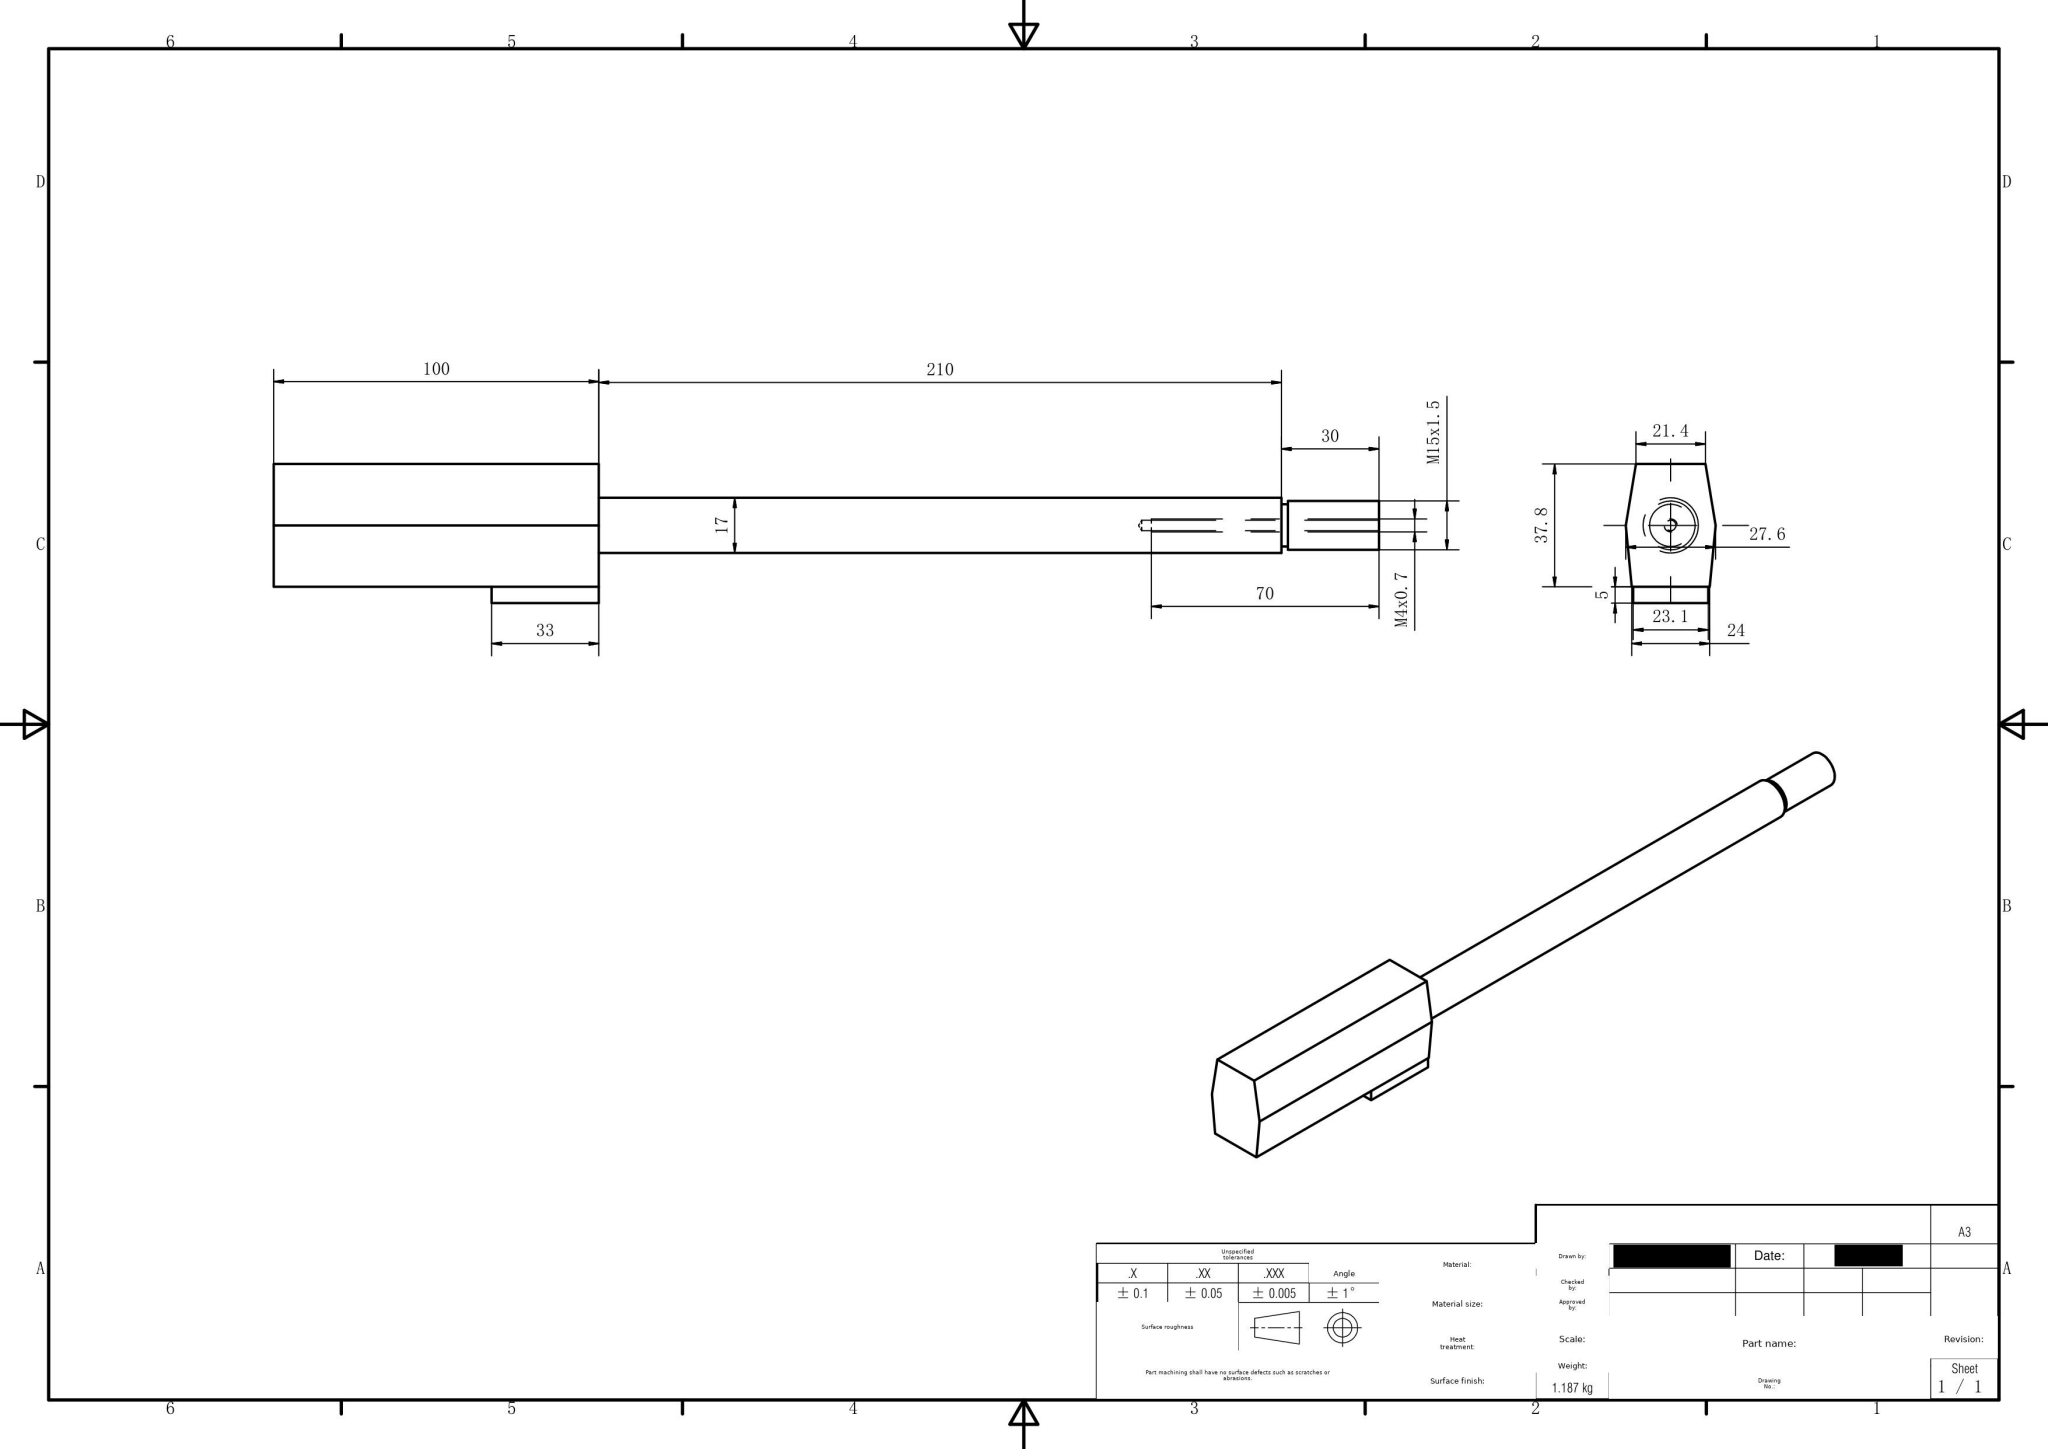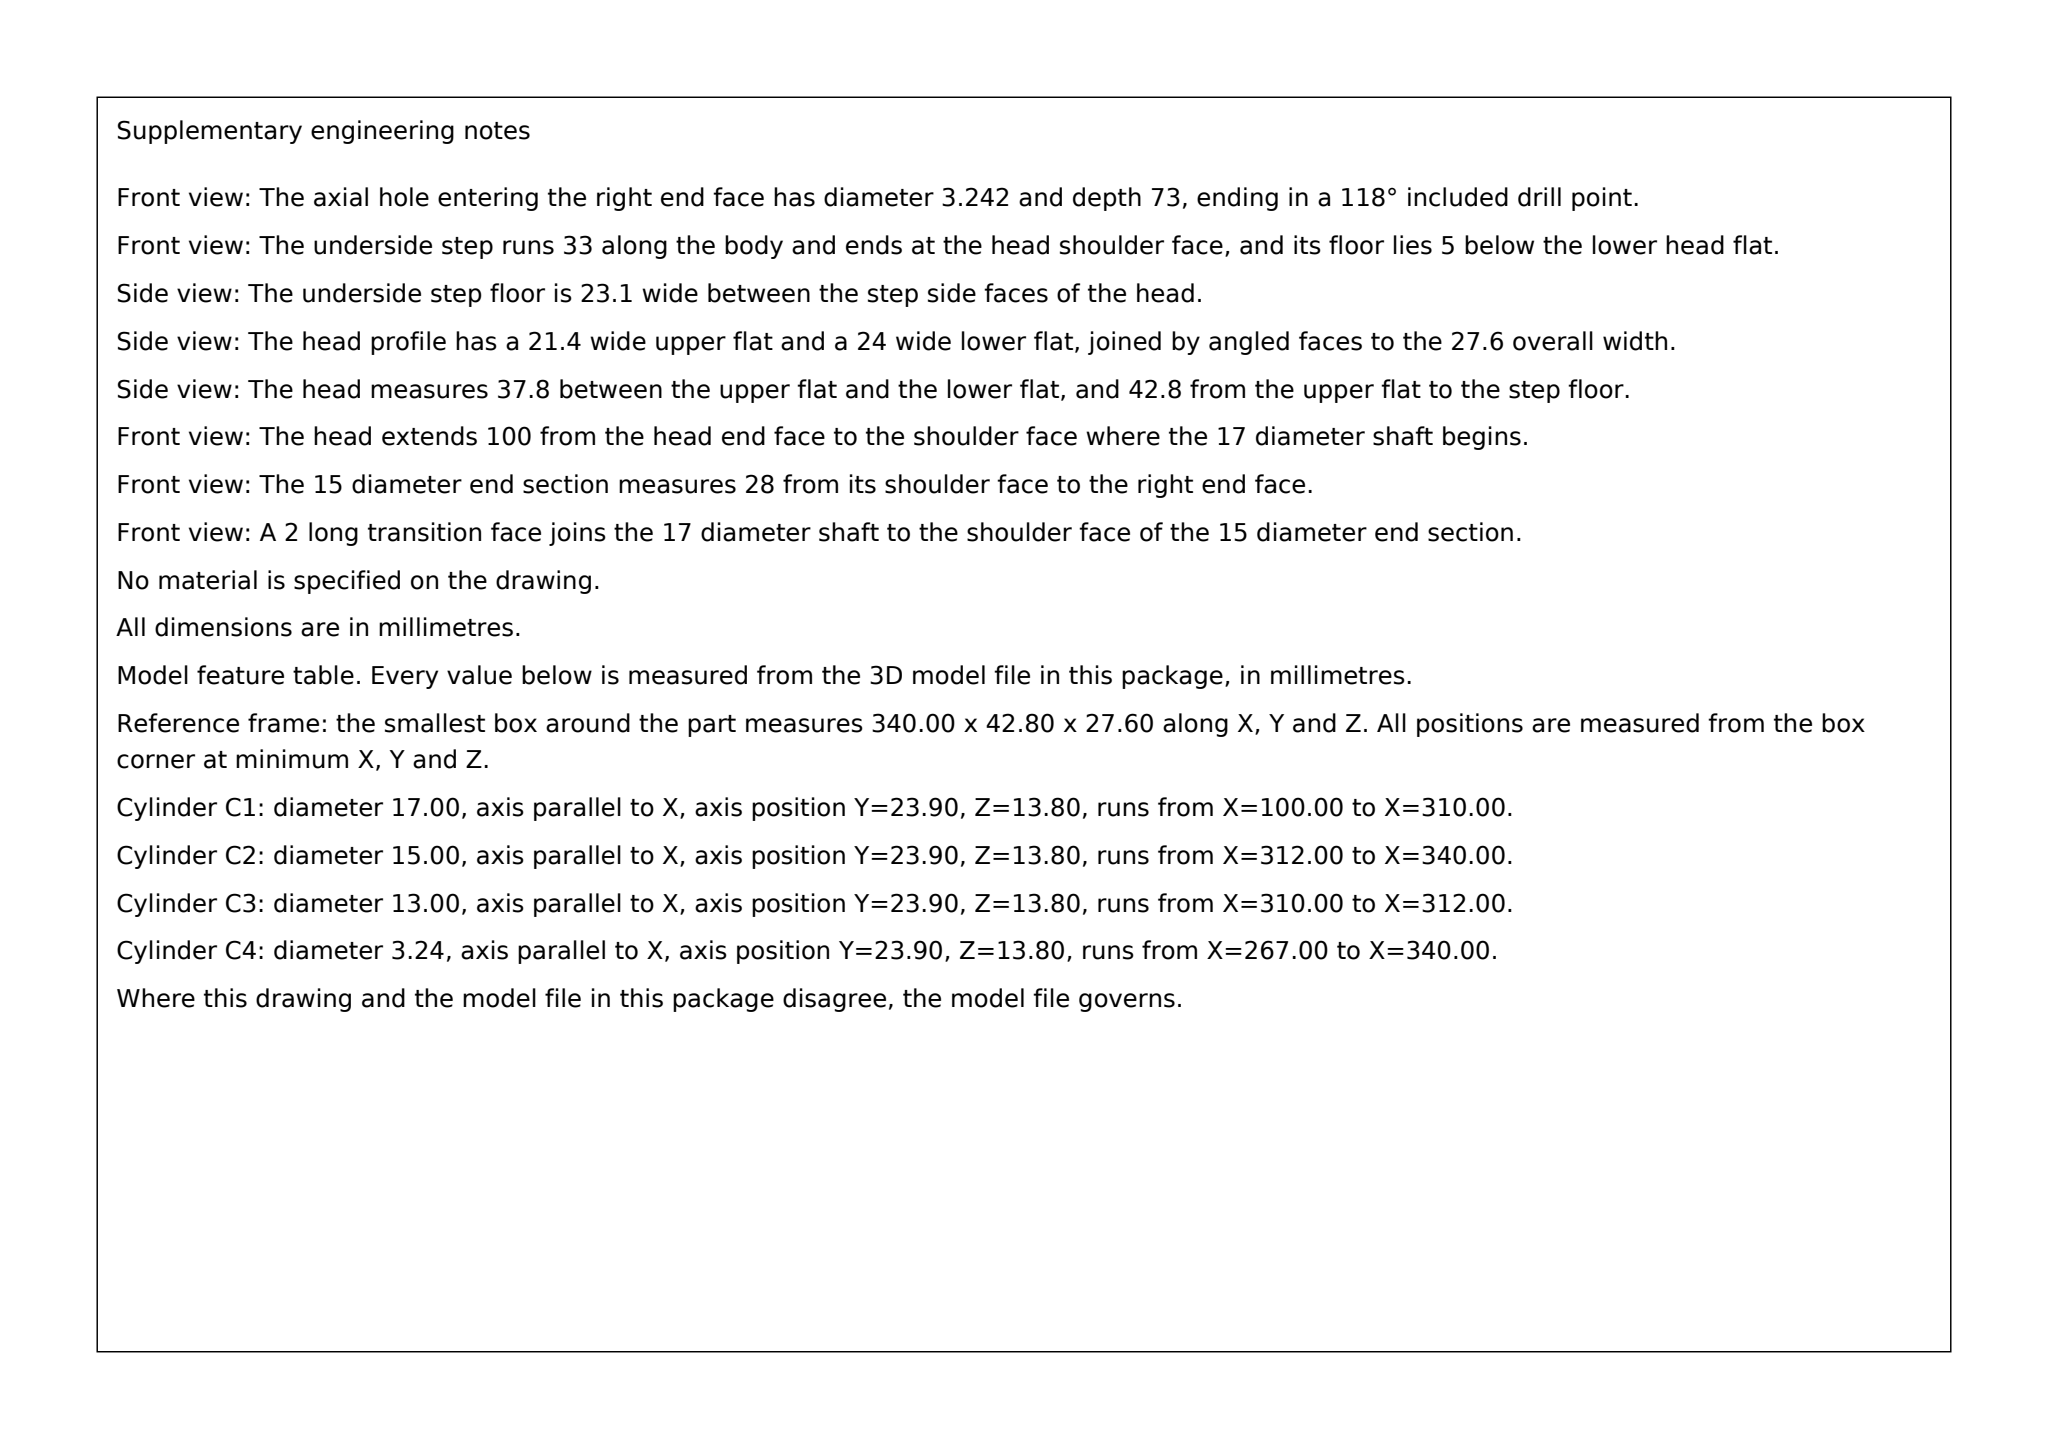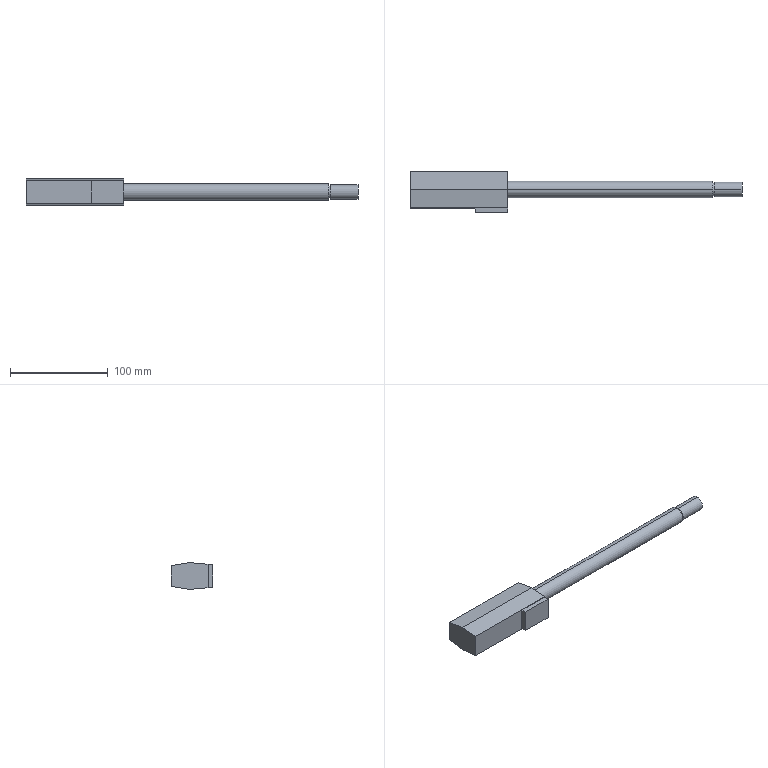Part | SolidWorks | mm | 1 solid | 25 faces | box 340 x 42.8 x 27.6 mm | volume 151152 mm3 | plane 15 | cylinder 8 | cone 2 | commonest cylinder face diameters 3.242 x2 13 x2 15 x2 17 x2
Drawing notes:
Ø13 x 2 WIDE RELIEF, FROM 310 TO 312 FROM HEAD BUTT END FACE (LH) | from the solid: cylinders[13.0,x,len 2.0]; axis_planes x=310.0 and x=312.0
HEAD OVERALL HEIGHT 42.8 FROM BOTTOM FACE (Y=0) TO TOP FACE (Y=42.8); SHAFT AXIS AT Y=23.9, Z=13.8 | from the solid: axis_planes y=0.0 and y=42.8; cylinders dia 17/15/13/3.242 axis x at [y=23.9, z=13.8]
HEAD BOTTOM STEP: 23.1 WIDE (Z=2.3 TO 25.4, SYMM ABOUT SHAFT AXIS Z=13.8) X 5 HIGH (Y=0 TO 5) X 33 LONG (X=67 TO 100 FROM HEAD BUTT END FACE X=0); 24 IS HEAD WIDTH AT Y=5 | from the solid: axis_planes y=0.0 extent x 67-100, z 2.3-25.4; z=2.3 and z=25.4 planes extent x 67-100, y 0-5; axis_plane x=67.0 extent y 0-5, z 2.3-25.4
TAP DRILL Ø3.242 THRU DEPTH 73 FROM THREADED END FACE X=340 (DRILL BOTTOM X=267, 118° POINT TO X=266), ON SHAFT AXIS Y=23.9 Z=13.8 | from the solid: hole/bore dia 3.24 axis x from 267.0 to 340.0 at [null,23.9,13.8]; cones included_angle 118.0 ref_dia 3.24 bbox_from [266.0,...]
M4x0.7 THD DP 70 FULL, TAP DRILL Ø3.24 DP 73 FROM M15x1.5 END | from the solid: hole/bore dia 3.24 along x from 267 to 340 (73 deep from end face x=340, which is the M15x1.5 end); 118° drill point at x=266-267; thread depth per existing 70 dim from same end face
build123d program:
from build123d import *

# Parameters (mm, degrees)
BOSS_EXTRUDE1_DEPTH      = 100
SKETCH2_W                = 33
SKETCH2_H                = 23.1
BOSS_EXTRUDE2_DEPTH      = 5
DRAFT1_ANGLE             = 5.44
M3_CLEARANCE_HOLE1_D     = 3.242
M3_CLEARANCE_HOLE1_DEPTH = 73
M3_CLEARANCE_HOLE1_TIP   = 0.974


with BuildPart() as part:
    # Sketch1 → Boss-Extrude1 (new body)
    with BuildSketch(Plane(origin=(100, 0, 0), x_dir=(0, 0, -1), z_dir=(1, 0, 0))):
        Polygon((-12, 10.974), (-12, -18.9), (12, -18.9), (12, 10.974), (10.7, 18.9), (-10.7, 18.9), align=None)
    extrude(amount=-BOSS_EXTRUDE1_DEPTH)

    # Sketch2 → Boss-Extrude2 (add)
    with BuildSketch(Plane.XZ.offset(18.9)):
        with Locations((83.5, 0)):
            Rectangle(SKETCH2_W, SKETCH2_H)
    extrude(amount=BOSS_EXTRUDE2_DEPTH)

    # Draft1
    draft1_faces = [part.faces().sort_by_distance(p)[0] for p in [
        (50, -3.963, 12),
        (50, -3.963, -12),
    ]]
    draft(draft1_faces, Plane(origin=(0, -18.9, 12), x_dir=(0, 0, -1), z_dir=(0, -1, 0)), DRAFT1_ANGLE)

    # Sketch3 → Revolve1 (revolve)
    with BuildSketch(Plane.XY, mode=Mode.PRIVATE) as revolve1_sk:
        Polygon((100, 8.5), (100, 0), (340, 0), (340, 7.5), (312, 7.5), (312, 6.5), (310, 6.5), (310, 8.5), align=None)
    revolve(revolve1_sk.sketch.rotate(Axis((100, 0, 0), (1, 0, 0)), 270), axis=Axis((100, 0, 0), (1, 0, 0)))

    # M3 Clearance Hole1
    with Locations(Plane(origin=(340, 0, 0), x_dir=(0, 0, -1), z_dir=(1, 0, 0))):
        with Locations((0, 0)):
            Hole(M3_CLEARANCE_HOLE1_D / 2, depth=M3_CLEARANCE_HOLE1_DEPTH)
            with Locations((0, 0, -(M3_CLEARANCE_HOLE1_DEPTH + M3_CLEARANCE_HOLE1_TIP / 2))):  # 118° drill point
                Cone(0, M3_CLEARANCE_HOLE1_D / 2, M3_CLEARANCE_HOLE1_TIP, mode=Mode.SUBTRACT)


solid = part.part
STEP:
#1=CARTESIAN_POINT('',(267.,0.,1.621));
#2=VERTEX_POINT('',#1);
#3=CARTESIAN_POINT('',(267.,0.,-1.621));
#4=VERTEX_POINT('',#3);
#5=CARTESIAN_POINT('',(267.,0.,0.));
#6=DIRECTION('',(1.,0.,0.));
#7=DIRECTION('',(0.,0.,-1.));
#8=AXIS2_PLACEMENT_3D('',#5,#6,#7);
#9=CIRCLE('',#8,1.621);
#10=EDGE_CURVE('',#2,#4,#9,.T.);
#11=ORIENTED_EDGE('',*,*,#10,.F.);
#12=CARTESIAN_POINT('',(340.,0.,1.621));
#13=VERTEX_POINT('',#12);
#14=CARTESIAN_POINT('',(340.,0.,1.621));
#15=DIRECTION('',(1.,0.,0.));
#16=VECTOR('',#15,1000.);
#17=LINE('',#14,#16);
#18=EDGE_CURVE('',#2,#13,#17,.T.);
#19=ORIENTED_EDGE('',*,*,#18,.T.);
#20=CARTESIAN_POINT('',(340.,0.,-1.621));
#21=VERTEX_POINT('',#20);
#22=CARTESIAN_POINT('',(340.,0.,0.));
#23=DIRECTION('',(1.,0.,0.));
#24=DIRECTION('',(0.,0.,-1.));
#25=AXIS2_PLACEMENT_3D('',#22,#23,#24);
#26=CIRCLE('',#25,1.621);
#27=EDGE_CURVE('',#13,#21,#26,.T.);
#28=ORIENTED_EDGE('',*,*,#27,.T.);
#29=CARTESIAN_POINT('',(340.,0.,-1.621));
#30=DIRECTION('',(1.,0.,0.));
#31=VECTOR('',#30,1000.);
#32=LINE('',#29,#31);
#33=EDGE_CURVE('',#4,#21,#32,.T.);
#34=ORIENTED_EDGE('',*,*,#33,.F.);
#35=EDGE_LOOP('',(#11,#19,#28,#34));
#36=FACE_OUTER_BOUND('',#35,.T.);
#37=CARTESIAN_POINT('',(340.,0.,0.));
#38=DIRECTION('',(1.,0.,0.));
#39=DIRECTION('',(0.,0.,-1.));
#40=AXIS2_PLACEMENT_3D('',#37,#38,#39);
#41=CYLINDRICAL_SURFACE('',#40,1.621);
#42=ADVANCED_FACE('',(#36),#41,.F.);
#43=CARTESIAN_POINT('',(266.026,-0.,0.));
#44=VERTEX_POINT('',#43);
#45=CARTESIAN_POINT('',(267.,0.,-1.621));
#46=DIRECTION('',(0.515,0.,-0.8572));
#47=VECTOR('',#46,1000.);
#48=LINE('',#45,#47);
#49=EDGE_CURVE('',#44,#4,#48,.T.);
#50=ORIENTED_EDGE('',*,*,#49,.F.);
#51=CARTESIAN_POINT('',(267.,0.,1.621));
#52=DIRECTION('',(0.515,0.,0.8572));
#53=VECTOR('',#52,1000.);
#54=LINE('',#51,#53);
#55=EDGE_CURVE('',#44,#2,#54,.T.);
#56=ORIENTED_EDGE('',*,*,#55,.T.);
#57=ORIENTED_EDGE('',*,*,#10,.T.);
#58=EDGE_LOOP('',(#50,#56,#57));
#59=FACE_OUTER_BOUND('',#58,.T.);
#60=CARTESIAN_POINT('',(267.,0.,0.));
#61=DIRECTION('',(1.,0.,0.));
#62=DIRECTION('',(0.,0.,-1.));
#63=AXIS2_PLACEMENT_3D('',#60,#61,#62);
#64=CONICAL_SURFACE('',#63,1.621,1.03);
#65=ADVANCED_FACE('',(#59),#64,.F.);
#66=CARTESIAN_POINT('',(310.,0.,-6.5));
#67=VERTEX_POINT('',#66);
#68=CARTESIAN_POINT('',(310.,0.,6.5));
#69=VERTEX_POINT('',#68);
#70=CARTESIAN_POINT('',(310.,0.,0.));
#71=DIRECTION('',(1.,0.,0.));
#72=DIRECTION('',(0.,0.,-1.));
#73=AXIS2_PLACEMENT_3D('',#70,#71,#72);
#74=CIRCLE('',#73,6.5);
#75=EDGE_CURVE('',#67,#69,#74,.T.);
#76=ORIENTED_EDGE('',*,*,#75,.T.);
#77=CARTESIAN_POINT('',(312.,0.,6.5));
#78=VERTEX_POINT('',#77);
#79=CARTESIAN_POINT('',(100.,0.,6.5));
#80=DIRECTION('',(1.,0.,0.));
#81=VECTOR('',#80,1000.);
#82=LINE('',#79,#81);
#83=EDGE_CURVE('',#69,#78,#82,.T.);
#84=ORIENTED_EDGE('',*,*,#83,.T.);
#85=CARTESIAN_POINT('',(312.,0.,-6.5));
#86=VERTEX_POINT('',#85);
#87=CARTESIAN_POINT('',(312.,0.,0.));
#88=DIRECTION('',(1.,0.,0.));
#89=DIRECTION('',(0.,0.,-1.));
#90=AXIS2_PLACEMENT_3D('',#87,#88,#89);
#91=CIRCLE('',#90,6.5);
#92=EDGE_CURVE('',#86,#78,#91,.T.);
#93=ORIENTED_EDGE('',*,*,#92,.F.);
#94=CARTESIAN_POINT('',(100.,0.,-6.5));
#95=DIRECTION('',(1.,0.,0.));
#96=VECTOR('',#95,1000.);
#97=LINE('',#94,#96);
#98=EDGE_CURVE('',#67,#86,#97,.T.);
#99=ORIENTED_EDGE('',*,*,#98,.F.);
#100=EDGE_LOOP('',(#76,#84,#93,#99));
#101=FACE_OUTER_BOUND('',#100,.T.);
#102=CARTESIAN_POINT('',(100.,0.,0.));
#103=DIRECTION('',(1.,0.,0.));
#104=DIRECTION('',(0.,0.,-1.));
#105=AXIS2_PLACEMENT_3D('',#102,#103,#104);
#106=CYLINDRICAL_SURFACE('',#105,6.5);
#107=ADVANCED_FACE('',(#101),#106,.T.);
#108=CARTESIAN_POINT('',(312.,0.,-7.5));
#109=VERTEX_POINT('',#108);
#110=CARTESIAN_POINT('',(312.,0.,7.5));
#111=VERTEX_POINT('',#110);
#112=CARTESIAN_POINT('',(312.,0.,0.));
#113=DIRECTION('',(1.,0.,0.));
#114=DIRECTION('',(0.,0.,-1.));
#115=AXIS2_PLACEMENT_3D('',#112,#113,#114);
#116=CIRCLE('',#115,7.5);
#117=EDGE_CURVE('',#109,#111,#116,.T.);
#118=ORIENTED_EDGE('',*,*,#117,.T.);
#119=CARTESIAN_POINT('',(340.,0.,7.5));
#120=VERTEX_POINT('',#119);
#121=CARTESIAN_POINT('',(100.,0.,7.5));
#122=DIRECTION('',(1.,0.,0.));
#123=VECTOR('',#122,1000.);
#124=LINE('',#121,#123);
#125=EDGE_CURVE('',#111,#120,#124,.T.);
#126=ORIENTED_EDGE('',*,*,#125,.T.);
#127=CARTESIAN_POINT('',(340.,0.,-7.5));
#128=VERTEX_POINT('',#127);
#129=CARTESIAN_POINT('',(340.,0.,0.));
#130=DIRECTION('',(1.,0.,0.));
#131=DIRECTION('',(0.,0.,-1.));
#132=AXIS2_PLACEMENT_3D('',#129,#130,#131);
#133=CIRCLE('',#132,7.5);
#134=EDGE_CURVE('',#128,#120,#133,.T.);
#135=ORIENTED_EDGE('',*,*,#134,.F.);
#136=CARTESIAN_POINT('',(100.,0.,-7.5));
#137=DIRECTION('',(1.,0.,0.));
#138=VECTOR('',#137,1000.);
#139=LINE('',#136,#138);
#140=EDGE_CURVE('',#109,#128,#139,.T.);
#141=ORIENTED_EDGE('',*,*,#140,.F.);
#142=EDGE_LOOP('',(#118,#126,#135,#141));
#143=FACE_OUTER_BOUND('',#142,.T.);
#144=CARTESIAN_POINT('',(100.,0.,0.));
#145=DIRECTION('',(1.,0.,0.));
#146=DIRECTION('',(0.,0.,-1.));
#147=AXIS2_PLACEMENT_3D('',#144,#145,#146);
#148=CYLINDRICAL_SURFACE('',#147,7.5);
#149=ADVANCED_FACE('',(#143),#148,.T.);
#150=CARTESIAN_POINT('',(100.,0.,-8.5));
#151=VERTEX_POINT('',#150);
#152=CARTESIAN_POINT('',(100.,0.,8.5));
#153=VERTEX_POINT('',#152);
#154=CARTESIAN_POINT('',(100.,0.,0.));
#155=DIRECTION('',(1.,0.,0.));
#156=DIRECTION('',(0.,0.,-1.));
#157=AXIS2_PLACEMENT_3D('',#154,#155,#156);
#158=CIRCLE('',#157,8.5);
#159=EDGE_CURVE('',#151,#153,#158,.T.);
#160=ORIENTED_EDGE('',*,*,#159,.T.);
#161=CARTESIAN_POINT('',(310.,0.,8.5));
#162=VERTEX_POINT('',#161);
#163=CARTESIAN_POINT('',(100.,0.,8.5));
#164=DIRECTION('',(1.,0.,0.));
#165=VECTOR('',#164,1000.);
#166=LINE('',#163,#165);
#167=EDGE_CURVE('',#153,#162,#166,.T.);
#168=ORIENTED_EDGE('',*,*,#167,.T.);
#169=CARTESIAN_POINT('',(310.,0.,-8.5));
#170=VERTEX_POINT('',#169);
#171=CARTESIAN_POINT('',(310.,0.,0.));
#172=DIRECTION('',(1.,0.,0.));
#173=DIRECTION('',(0.,0.,-1.));
#174=AXIS2_PLACEMENT_3D('',#171,#172,#173);
#175=CIRCLE('',#174,8.5);
#176=EDGE_CURVE('',#170,#162,#175,.T.);
#177=ORIENTED_EDGE('',*,*,#176,.F.);
#178=CARTESIAN_POINT('',(100.,0.,-8.5));
#179=DIRECTION('',(1.,0.,0.));
#180=VECTOR('',#179,1000.);
#181=LINE('',#178,#180);
#182=EDGE_CURVE('',#151,#170,#181,.T.);
#183=ORIENTED_EDGE('',*,*,#182,.F.);
#184=EDGE_LOOP('',(#160,#168,#177,#183));
#185=FACE_OUTER_BOUND('',#184,.T.);
#186=CARTESIAN_POINT('',(100.,0.,0.));
#187=DIRECTION('',(1.,0.,0.));
#188=DIRECTION('',(0.,0.,-1.));
#189=AXIS2_PLACEMENT_3D('',#186,#187,#188);
#190=CYLINDRICAL_SURFACE('',#189,8.5);
#191=ADVANCED_FACE('',(#185),#190,.T.);
#192=CARTESIAN_POINT('',(100.,18.9,10.7));
#193=VERTEX_POINT('',#192);
#194=CARTESIAN_POINT('',(100.,-0.,13.8));
#195=VERTEX_POINT('',#194);
#196=CARTESIAN_POINT('',(100.,18.9,10.7));
#197=DIRECTION('',(0.,-0.9868,0.1619));
#198=VECTOR('',#197,1000.);
#199=LINE('',#196,#198);
#200=EDGE_CURVE('',#193,#195,#199,.T.);
#201=ORIENTED_EDGE('',*,*,#200,.F.);
#202=CARTESIAN_POINT('',(0.,18.9,10.7));
#203=VERTEX_POINT('',#202);
#204=CARTESIAN_POINT('',(0.,18.9,10.7));
#205=DIRECTION('',(1.,0.,0.));
#206=VECTOR('',#205,1000.);
#207=LINE('',#204,#206);
#208=EDGE_CURVE('',#203,#193,#207,.T.);
#209=ORIENTED_EDGE('',*,*,#208,.F.);
#210=CARTESIAN_POINT('',(0.,-0.,13.8));
#211=VERTEX_POINT('',#210);
#212=CARTESIAN_POINT('',(0.,18.9,10.7));
#213=DIRECTION('',(0.,-0.9868,0.1619));
#214=VECTOR('',#213,1000.);
#215=LINE('',#212,#214);
#216=EDGE_CURVE('',#203,#211,#215,.T.);
#217=ORIENTED_EDGE('',*,*,#216,.T.);
#218=CARTESIAN_POINT('',(0.,-0.,13.8));
#219=DIRECTION('',(1.,0.,0.));
#220=VECTOR('',#219,1000.);
#221=LINE('',#218,#220);
#222=EDGE_CURVE('',#211,#195,#221,.T.);
#223=ORIENTED_EDGE('',*,*,#222,.T.);
#224=EDGE_LOOP('',(#201,#209,#217,#223));
#225=FACE_OUTER_BOUND('',#224,.T.);
#226=CARTESIAN_POINT('',(0.,18.9,10.7));
#227=DIRECTION('',(0.,0.1619,0.9868));
#228=DIRECTION('',(0.,-0.9868,0.1619));
#229=AXIS2_PLACEMENT_3D('',#226,#227,#228);
#230=PLANE('',#229);
#231=ADVANCED_FACE('',(#225),#230,.T.);
#232=CARTESIAN_POINT('',(100.,18.9,-10.7));
#233=VERTEX_POINT('',#232);
#234=CARTESIAN_POINT('',(100.,18.9,-10.7));
#235=DIRECTION('',(0.,-0.,1.));
#236=VECTOR('',#235,1000.);
#237=LINE('',#234,#236);
#238=EDGE_CURVE('',#233,#193,#237,.T.);
#239=ORIENTED_EDGE('',*,*,#238,.F.);
#240=CARTESIAN_POINT('',(0.,18.9,-10.7));
#241=VERTEX_POINT('',#240);
#242=CARTESIAN_POINT('',(0.,18.9,-10.7));
#243=DIRECTION('',(1.,0.,0.));
#244=VECTOR('',#243,1000.);
#245=LINE('',#242,#244);
#246=EDGE_CURVE('',#241,#233,#245,.T.);
#247=ORIENTED_EDGE('',*,*,#246,.F.);
#248=CARTESIAN_POINT('',(0.,18.9,-10.7));
#249=DIRECTION('',(0.,-0.,1.));
#250=VECTOR('',#249,1000.);
#251=LINE('',#248,#250);
#252=EDGE_CURVE('',#241,#203,#251,.T.);
#253=ORIENTED_EDGE('',*,*,#252,.T.);
#254=ORIENTED_EDGE('',*,*,#208,.T.);
#255=EDGE_LOOP('',(#239,#247,#253,#254));
#256=FACE_OUTER_BOUND('',#255,.T.);
#257=CARTESIAN_POINT('',(0.,18.9,-10.7));
#258=DIRECTION('',(0.,1.,0.));
#259=DIRECTION('',(0.,-0.,1.));
#260=AXIS2_PLACEMENT_3D('',#257,#258,#259);
#261=PLANE('',#260);
#262=ADVANCED_FACE('',(#256),#261,.T.);
#263=CARTESIAN_POINT('',(100.,-0.,-13.8));
#264=VERTEX_POINT('',#263);
#265=CARTESIAN_POINT('',(100.,10.974,-12.));
#266=DIRECTION('',(0.,0.9868,0.1619));
#267=VECTOR('',#266,1000.);
#268=LINE('',#265,#267);
#269=EDGE_CURVE('',#264,#233,#268,.T.);
#270=ORIENTED_EDGE('',*,*,#269,.F.);
#271=CARTESIAN_POINT('',(0.,-0.,-13.8));
#272=VERTEX_POINT('',#271);
#273=CARTESIAN_POINT('',(0.,-0.,-13.8));
#274=DIRECTION('',(1.,0.,0.));
#275=VECTOR('',#274,1000.);
#276=LINE('',#273,#275);
#277=EDGE_CURVE('',#272,#264,#276,.T.);
#278=ORIENTED_EDGE('',*,*,#277,.F.);
#279=CARTESIAN_POINT('',(0.,10.974,-12.));
#280=DIRECTION('',(0.,0.9868,0.1619));
#281=VECTOR('',#280,1000.);
#282=LINE('',#279,#281);
#283=EDGE_CURVE('',#272,#241,#282,.T.);
#284=ORIENTED_EDGE('',*,*,#283,.T.);
#285=ORIENTED_EDGE('',*,*,#246,.T.);
#286=EDGE_LOOP('',(#270,#278,#284,#285));
#287=FACE_OUTER_BOUND('',#286,.T.);
#288=CARTESIAN_POINT('',(0.,10.974,-12.));
#289=DIRECTION('',(0.,0.1619,-0.9868));
#290=DIRECTION('',(0.,0.9868,0.1619));
#291=AXIS2_PLACEMENT_3D('',#288,#289,#290);
#292=PLANE('',#291);
#293=ADVANCED_FACE('',(#287),#292,.T.);
#294=CARTESIAN_POINT('',(100.,-18.9,-12.));
#295=VERTEX_POINT('',#294);
#296=CARTESIAN_POINT('',(100.,-1.302,-13.676));
#297=DIRECTION('',(0.,0.9955,-0.09481));
#298=VECTOR('',#297,1000.);
#299=LINE('',#296,#298);
#300=EDGE_CURVE('',#295,#264,#299,.T.);
#301=ORIENTED_EDGE('',*,*,#300,.F.);
#302=CARTESIAN_POINT('',(0.,-18.9,-12.));
#303=VERTEX_POINT('',#302);
#304=CARTESIAN_POINT('',(0.,-18.9,-12.));
#305=DIRECTION('',(1.,0.,0.));
#306=VECTOR('',#305,1000.);
#307=LINE('',#304,#306);
#308=EDGE_CURVE('',#303,#295,#307,.T.);
#309=ORIENTED_EDGE('',*,*,#308,.F.);
#310=CARTESIAN_POINT('',(0.,-1.302,-13.676));
#311=DIRECTION('',(0.,0.9955,-0.09481));
#312=VECTOR('',#311,1000.);
#313=LINE('',#310,#312);
#314=EDGE_CURVE('',#303,#272,#313,.T.);
#315=ORIENTED_EDGE('',*,*,#314,.T.);
#316=ORIENTED_EDGE('',*,*,#277,.T.);
#317=EDGE_LOOP('',(#301,#309,#315,#316));
#318=FACE_OUTER_BOUND('',#317,.T.);
#319=CARTESIAN_POINT('',(0.,-18.9,-12.));
#320=DIRECTION('',(0.,-0.09481,-0.9955));
#321=DIRECTION('',(0.,0.9955,-0.09481));
#322=AXIS2_PLACEMENT_3D('',#319,#320,#321);
#323=PLANE('',#322);
#324=ADVANCED_FACE('',(#318),#323,.T.);
#325=CARTESIAN_POINT('',(67.,-18.9,-11.55));
#326=VERTEX_POINT('',#325);
#327=CARTESIAN_POINT('',(100.,-18.9,-11.55));
#328=VERTEX_POINT('',#327);
#329=CARTESIAN_POINT('',(100.,-18.9,-11.55));
#330=DIRECTION('',(1.,0.,0.));
#331=VECTOR('',#330,1000.);
#332=LINE('',#329,#331);
#333=EDGE_CURVE('',#326,#328,#332,.T.);
#334=ORIENTED_EDGE('',*,*,#333,.F.);
#335=CARTESIAN_POINT('',(67.,-18.9,11.55));
#336=VERTEX_POINT('',#335);
#337=CARTESIAN_POINT('',(67.,-18.9,-11.55));
#338=DIRECTION('',(0.,0.,-1.));
#339=VECTOR('',#338,1000.);
#340=LINE('',#337,#339);
#341=EDGE_CURVE('',#336,#326,#340,.T.);
#342=ORIENTED_EDGE('',*,*,#341,.F.);
#343=CARTESIAN_POINT('',(100.,-18.9,11.55));
#344=VERTEX_POINT('',#343);
#345=CARTESIAN_POINT('',(67.,-18.9,11.55));
#346=DIRECTION('',(-1.,0.,0.));
#347=VECTOR('',#346,1000.);
#348=LINE('',#345,#347);
#349=EDGE_CURVE('',#344,#336,#348,.T.);
#350=ORIENTED_EDGE('',*,*,#349,.F.);
#351=CARTESIAN_POINT('',(100.,-18.9,12.));
#352=VERTEX_POINT('',#351);
#353=CARTESIAN_POINT('',(100.,-18.9,12.));
#354=DIRECTION('',(0.,0.,-1.));
#355=VECTOR('',#354,1000.);
#356=LINE('',#353,#355);
#357=EDGE_CURVE('',#352,#344,#356,.T.);
#358=ORIENTED_EDGE('',*,*,#357,.F.);
#359=CARTESIAN_POINT('',(0.,-18.9,12.));
#360=VERTEX_POINT('',#359);
#361=CARTESIAN_POINT('',(0.,-18.9,12.));
#362=DIRECTION('',(1.,0.,0.));
#363=VECTOR('',#362,1000.);
#364=LINE('',#361,#363);
#365=EDGE_CURVE('',#360,#352,#364,.T.);
#366=ORIENTED_EDGE('',*,*,#365,.F.);
#367=CARTESIAN_POINT('',(0.,-18.9,12.));
#368=DIRECTION('',(0.,0.,-1.));
#369=VECTOR('',#368,1000.);
#370=LINE('',#367,#369);
#371=EDGE_CURVE('',#360,#303,#370,.T.);
#372=ORIENTED_EDGE('',*,*,#371,.T.);
#373=ORIENTED_EDGE('',*,*,#308,.T.);
#374=CARTESIAN_POINT('',(100.,-18.9,12.));
#375=DIRECTION('',(0.,0.,-1.));
#376=VECTOR('',#375,1000.);
#377=LINE('',#374,#376);
#378=EDGE_CURVE('',#328,#295,#377,.T.);
#379=ORIENTED_EDGE('',*,*,#378,.F.);
#380=EDGE_LOOP('',(#334,#342,#350,#358,#366,#372,#373,#379));
#381=FACE_OUTER_BOUND('',#380,.T.);
#382=CARTESIAN_POINT('',(0.,-18.9,12.));
#383=DIRECTION('',(0.,-1.,-0.));
#384=DIRECTION('',(0.,0.,-1.));
#385=AXIS2_PLACEMENT_3D('',#382,#383,#384);
#386=PLANE('',#385);
#387=ADVANCED_FACE('',(#381),#386,.T.);
#388=CARTESIAN_POINT('',(100.,-1.302,13.676));
#389=DIRECTION('',(0.,-0.9955,-0.09481));
#390=VECTOR('',#389,1000.);
#391=LINE('',#388,#390);
#392=EDGE_CURVE('',#195,#352,#391,.T.);
#393=ORIENTED_EDGE('',*,*,#392,.F.);
#394=ORIENTED_EDGE('',*,*,#222,.F.);
#395=CARTESIAN_POINT('',(0.,-1.302,13.676));
#396=DIRECTION('',(0.,-0.9955,-0.09481));
#397=VECTOR('',#396,1000.);
#398=LINE('',#395,#397);
#399=EDGE_CURVE('',#211,#360,#398,.T.);
#400=ORIENTED_EDGE('',*,*,#399,.T.);
#401=ORIENTED_EDGE('',*,*,#365,.T.);
#402=EDGE_LOOP('',(#393,#394,#400,#401));
#403=FACE_OUTER_BOUND('',#402,.T.);
#404=CARTESIAN_POINT('',(0.,-18.9,12.));
#405=DIRECTION('',(0.,-0.09481,0.9955));
#406=DIRECTION('',(0.,-0.9955,-0.09481));
#407=AXIS2_PLACEMENT_3D('',#404,#405,#406);
#408=PLANE('',#407);
#409=ADVANCED_FACE('',(#403),#408,.T.);
#410=ORIENTED_EDGE('',*,*,#216,.F.);
#411=ORIENTED_EDGE('',*,*,#252,.F.);
#412=ORIENTED_EDGE('',*,*,#283,.F.);
#413=ORIENTED_EDGE('',*,*,#314,.F.);
#414=ORIENTED_EDGE('',*,*,#371,.F.);
#415=ORIENTED_EDGE('',*,*,#399,.F.);
#416=EDGE_LOOP('',(#410,#411,#412,#413,#414,#415));
#417=FACE_OUTER_BOUND('',#416,.T.);
#418=CARTESIAN_POINT('',(0.,0.,0.));
#419=DIRECTION('',(1.,0.,0.));
#420=DIRECTION('',(0.,0.,-1.));
#421=AXIS2_PLACEMENT_3D('',#418,#419,#420);
#422=PLANE('',#421);
#423=ADVANCED_FACE('',(#417),#422,.F.);
#424=ORIENTED_EDGE('',*,*,#159,.F.);
#425=CARTESIAN_POINT('',(100.,0.,0.));
#426=DIRECTION('',(1.,0.,0.));
#427=DIRECTION('',(0.,0.,-1.));
#428=AXIS2_PLACEMENT_3D('',#425,#426,#427);
#429=CIRCLE('',#428,8.5);
#430=EDGE_CURVE('',#153,#151,#429,.T.);
#431=ORIENTED_EDGE('',*,*,#430,.F.);
#432=EDGE_LOOP('',(#424,#431));
#433=FACE_BOUND('',#432,.T.);
#434=ORIENTED_EDGE('',*,*,#200,.T.);
#435=ORIENTED_EDGE('',*,*,#392,.T.);
#436=ORIENTED_EDGE('',*,*,#357,.T.);
#437=CARTESIAN_POINT('',(100.,-23.9,11.55));
#438=VERTEX_POINT('',#437);
#439=CARTESIAN_POINT('',(100.,-23.9,11.55));
#440=DIRECTION('',(0.,1.,0.));
#441=VECTOR('',#440,1000.);
#442=LINE('',#439,#441);
#443=EDGE_CURVE('',#438,#344,#442,.T.);
#444=ORIENTED_EDGE('',*,*,#443,.F.);
#445=CARTESIAN_POINT('',(100.,-23.9,-11.55));
#446=VERTEX_POINT('',#445);
#447=CARTESIAN_POINT('',(100.,-23.9,11.55));
#448=DIRECTION('',(0.,0.,1.));
#449=VECTOR('',#448,1000.);
#450=LINE('',#447,#449);
#451=EDGE_CURVE('',#446,#438,#450,.T.);
#452=ORIENTED_EDGE('',*,*,#451,.F.);
#453=CARTESIAN_POINT('',(100.,-23.9,-11.55));
#454=DIRECTION('',(0.,1.,0.));
#455=VECTOR('',#454,1000.);
#456=LINE('',#453,#455);
#457=EDGE_CURVE('',#446,#328,#456,.T.);
#458=ORIENTED_EDGE('',*,*,#457,.T.);
#459=ORIENTED_EDGE('',*,*,#378,.T.);
#460=ORIENTED_EDGE('',*,*,#300,.T.);
#461=ORIENTED_EDGE('',*,*,#269,.T.);
#462=ORIENTED_EDGE('',*,*,#238,.T.);
#463=EDGE_LOOP('',(#434,#435,#436,#444,#452,#458,#459,#460,#461,#462));
#464=FACE_OUTER_BOUND('',#463,.T.);
#465=CARTESIAN_POINT('',(100.,0.,0.));
#466=DIRECTION('',(1.,0.,0.));
#467=DIRECTION('',(0.,0.,-1.));
#468=AXIS2_PLACEMENT_3D('',#465,#466,#467);
#469=PLANE('',#468);
#470=ADVANCED_FACE('',(#433,#464),#469,.T.);
#471=ORIENTED_EDGE('',*,*,#333,.T.);
#472=ORIENTED_EDGE('',*,*,#457,.F.);
#473=CARTESIAN_POINT('',(67.,-23.9,-11.55));
#474=VERTEX_POINT('',#473);
#475=CARTESIAN_POINT('',(100.,-23.9,-11.55));
#476=DIRECTION('',(1.,0.,0.));
#477=VECTOR('',#476,1000.);
#478=LINE('',#475,#477);
#479=EDGE_CURVE('',#474,#446,#478,.T.);
#480=ORIENTED_EDGE('',*,*,#479,.F.);
#481=CARTESIAN_POINT('',(67.,-23.9,-11.55));
#482=DIRECTION('',(0.,1.,0.));
#483=VECTOR('',#482,1000.);
#484=LINE('',#481,#483);
#485=EDGE_CURVE('',#474,#326,#484,.T.);
#486=ORIENTED_EDGE('',*,*,#485,.T.);
#487=EDGE_LOOP('',(#471,#472,#480,#486));
#488=FACE_OUTER_BOUND('',#487,.T.);
#489=CARTESIAN_POINT('',(100.,-23.9,-11.55));
#490=DIRECTION('',(0.,-0.,1.));
#491=DIRECTION('',(0.,-1.,-0.));
#492=AXIS2_PLACEMENT_3D('',#489,#490,#491);
#493=PLANE('',#492);
#494=ADVANCED_FACE('',(#488),#493,.F.);
#495=ORIENTED_EDGE('',*,*,#349,.T.);
#496=CARTESIAN_POINT('',(67.,-23.9,11.55));
#497=VERTEX_POINT('',#496);
#498=CARTESIAN_POINT('',(67.,-23.9,11.55));
#499=DIRECTION('',(0.,1.,0.));
#500=VECTOR('',#499,1000.);
#501=LINE('',#498,#500);
#502=EDGE_CURVE('',#497,#336,#501,.T.);
#503=ORIENTED_EDGE('',*,*,#502,.F.);
#504=CARTESIAN_POINT('',(67.,-23.9,11.55));
#505=DIRECTION('',(-1.,0.,0.));
#506=VECTOR('',#505,1000.);
#507=LINE('',#504,#506);
#508=EDGE_CURVE('',#438,#497,#507,.T.);
#509=ORIENTED_EDGE('',*,*,#508,.F.);
#510=ORIENTED_EDGE('',*,*,#443,.T.);
#511=EDGE_LOOP('',(#495,#503,#509,#510));
#512=FACE_OUTER_BOUND('',#511,.T.);
#513=CARTESIAN_POINT('',(67.,-23.9,11.55));
#514=DIRECTION('',(0.,0.,-1.));
#515=DIRECTION('',(0.,1.,0.));
#516=AXIS2_PLACEMENT_3D('',#513,#514,#515);
#517=PLANE('',#516);
#518=ADVANCED_FACE('',(#512),#517,.F.);
#519=ORIENTED_EDGE('',*,*,#341,.T.);
#520=ORIENTED_EDGE('',*,*,#485,.F.);
#521=CARTESIAN_POINT('',(67.,-23.9,-11.55));
#522=DIRECTION('',(0.,0.,-1.));
#523=VECTOR('',#522,1000.);
#524=LINE('',#521,#523);
#525=EDGE_CURVE('',#497,#474,#524,.T.);
#526=ORIENTED_EDGE('',*,*,#525,.F.);
#527=ORIENTED_EDGE('',*,*,#502,.T.);
#528=EDGE_LOOP('',(#519,#520,#526,#527));
#529=FACE_OUTER_BOUND('',#528,.T.);
#530=CARTESIAN_POINT('',(67.,-23.9,-11.55));
#531=DIRECTION('',(1.,0.,0.));
#532=DIRECTION('',(0.,0.,-1.));
#533=AXIS2_PLACEMENT_3D('',#530,#531,#532);
#534=PLANE('',#533);
#535=ADVANCED_FACE('',(#529),#534,.F.);
#536=ORIENTED_EDGE('',*,*,#479,.T.);
#537=ORIENTED_EDGE('',*,*,#451,.T.);
#538=ORIENTED_EDGE('',*,*,#508,.T.);
#539=ORIENTED_EDGE('',*,*,#525,.T.);
#540=EDGE_LOOP('',(#536,#537,#538,#539));
#541=FACE_OUTER_BOUND('',#540,.T.);
#542=CARTESIAN_POINT('',(0.,-23.9,-0.));
#543=DIRECTION('',(0.,1.,0.));
#544=DIRECTION('',(0.,0.,1.));
#545=AXIS2_PLACEMENT_3D('',#542,#543,#544);
#546=PLANE('',#545);
#547=ADVANCED_FACE('',(#541),#546,.F.);
#548=ORIENTED_EDGE('',*,*,#167,.F.);
#549=ORIENTED_EDGE('',*,*,#430,.T.);
#550=ORIENTED_EDGE('',*,*,#182,.T.);
#551=CARTESIAN_POINT('',(310.,0.,0.));
#552=DIRECTION('',(1.,0.,0.));
#553=DIRECTION('',(0.,0.,-1.));
#554=AXIS2_PLACEMENT_3D('',#551,#552,#553);
#555=CIRCLE('',#554,8.5);
#556=EDGE_CURVE('',#162,#170,#555,.T.);
#557=ORIENTED_EDGE('',*,*,#556,.F.);
#558=EDGE_LOOP('',(#548,#549,#550,#557));
#559=FACE_OUTER_BOUND('',#558,.T.);
#560=CARTESIAN_POINT('',(100.,0.,0.));
#561=DIRECTION('',(1.,0.,0.));
#562=DIRECTION('',(0.,0.,-1.));
#563=AXIS2_PLACEMENT_3D('',#560,#561,#562);
#564=CYLINDRICAL_SURFACE('',#563,8.5);
#565=ADVANCED_FACE('',(#559),#564,.T.);
#566=CARTESIAN_POINT('',(340.,0.,0.));
#567=DIRECTION('',(1.,0.,0.));
#568=DIRECTION('',(0.,0.,-1.));
#569=AXIS2_PLACEMENT_3D('',#566,#567,#568);
#570=CIRCLE('',#569,1.621);
#571=EDGE_CURVE('',#21,#13,#570,.T.);
#572=ORIENTED_EDGE('',*,*,#571,.F.);
#573=ORIENTED_EDGE('',*,*,#27,.F.);
#574=EDGE_LOOP('',(#572,#573));
#575=FACE_BOUND('',#574,.T.);
#576=ORIENTED_EDGE('',*,*,#134,.T.);
#577=CARTESIAN_POINT('',(340.,0.,0.));
#578=DIRECTION('',(1.,0.,0.));
#579=DIRECTION('',(0.,0.,-1.));
#580=AXIS2_PLACEMENT_3D('',#577,#578,#579);
#581=CIRCLE('',#580,7.5);
#582=EDGE_CURVE('',#120,#128,#581,.T.);
#583=ORIENTED_EDGE('',*,*,#582,.T.);
#584=EDGE_LOOP('',(#576,#583));
#585=FACE_OUTER_BOUND('',#584,.T.);
#586=CARTESIAN_POINT('',(340.,0.,0.));
#587=DIRECTION('',(1.,0.,0.));
#588=DIRECTION('',(0.,0.,-1.));
#589=AXIS2_PLACEMENT_3D('',#586,#587,#588);
#590=PLANE('',#589);
#591=ADVANCED_FACE('',(#575,#585),#590,.T.);
#592=ORIENTED_EDGE('',*,*,#125,.F.);
#593=CARTESIAN_POINT('',(312.,0.,0.));
#594=DIRECTION('',(1.,0.,0.));
#595=DIRECTION('',(0.,0.,-1.));
#596=AXIS2_PLACEMENT_3D('',#593,#594,#595);
#597=CIRCLE('',#596,7.5);
#598=EDGE_CURVE('',#111,#109,#597,.T.);
#599=ORIENTED_EDGE('',*,*,#598,.T.);
#600=ORIENTED_EDGE('',*,*,#140,.T.);
#601=ORIENTED_EDGE('',*,*,#582,.F.);
#602=EDGE_LOOP('',(#592,#599,#600,#601));
#603=FACE_OUTER_BOUND('',#602,.T.);
#604=CARTESIAN_POINT('',(100.,0.,0.));
#605=DIRECTION('',(1.,0.,0.));
#606=DIRECTION('',(0.,0.,-1.));
#607=AXIS2_PLACEMENT_3D('',#604,#605,#606);
#608=CYLINDRICAL_SURFACE('',#607,7.5);
#609=ADVANCED_FACE('',(#603),#608,.T.);
#610=ORIENTED_EDGE('',*,*,#92,.T.);
#611=CARTESIAN_POINT('',(312.,0.,0.));
#612=DIRECTION('',(1.,0.,0.));
#613=DIRECTION('',(0.,0.,-1.));
#614=AXIS2_PLACEMENT_3D('',#611,#612,#613);
#615=CIRCLE('',#614,6.5);
#616=EDGE_CURVE('',#78,#86,#615,.T.);
#617=ORIENTED_EDGE('',*,*,#616,.T.);
#618=EDGE_LOOP('',(#610,#617));
#619=FACE_BOUND('',#618,.T.);
#620=ORIENTED_EDGE('',*,*,#117,.F.);
#621=ORIENTED_EDGE('',*,*,#598,.F.);
#622=EDGE_LOOP('',(#620,#621));
#623=FACE_OUTER_BOUND('',#622,.T.);
#624=CARTESIAN_POINT('',(312.,7.5,0.));
#625=DIRECTION('',(-1.,0.,0.));
#626=DIRECTION('',(0.,0.,1.));
#627=AXIS2_PLACEMENT_3D('',#624,#625,#626);
#628=PLANE('',#627);
#629=ADVANCED_FACE('',(#619,#623),#628,.T.);
#630=ORIENTED_EDGE('',*,*,#83,.F.);
#631=CARTESIAN_POINT('',(310.,0.,0.));
#632=DIRECTION('',(1.,0.,0.));
#633=DIRECTION('',(0.,0.,-1.));
#634=AXIS2_PLACEMENT_3D('',#631,#632,#633);
#635=CIRCLE('',#634,6.5);
#636=EDGE_CURVE('',#69,#67,#635,.T.);
#637=ORIENTED_EDGE('',*,*,#636,.T.);
#638=ORIENTED_EDGE('',*,*,#98,.T.);
#639=ORIENTED_EDGE('',*,*,#616,.F.);
#640=EDGE_LOOP('',(#630,#637,#638,#639));
#641=FACE_OUTER_BOUND('',#640,.T.);
#642=CARTESIAN_POINT('',(100.,0.,0.));
#643=DIRECTION('',(1.,0.,0.));
#644=DIRECTION('',(0.,0.,-1.));
#645=AXIS2_PLACEMENT_3D('',#642,#643,#644);
#646=CYLINDRICAL_SURFACE('',#645,6.5);
#647=ADVANCED_FACE('',(#641),#646,.T.);
#648=ORIENTED_EDGE('',*,*,#176,.T.);
#649=ORIENTED_EDGE('',*,*,#556,.T.);
#650=EDGE_LOOP('',(#648,#649));
#651=FACE_OUTER_BOUND('',#650,.T.);
#652=ORIENTED_EDGE('',*,*,#75,.F.);
#653=ORIENTED_EDGE('',*,*,#636,.F.);
#654=EDGE_LOOP('',(#652,#653));
#655=FACE_BOUND('',#654,.T.);
#656=CARTESIAN_POINT('',(310.,6.5,0.));
#657=DIRECTION('',(1.,0.,0.));
#658=DIRECTION('',(0.,0.,-1.));
#659=AXIS2_PLACEMENT_3D('',#656,#657,#658);
#660=PLANE('',#659);
#661=ADVANCED_FACE('',(#651,#655),#660,.T.);
#662=ORIENTED_EDGE('',*,*,#55,.F.);
#663=ORIENTED_EDGE('',*,*,#49,.T.);
#664=CARTESIAN_POINT('',(267.,0.,0.));
#665=DIRECTION('',(1.,0.,0.));
#666=DIRECTION('',(0.,0.,-1.));
#667=AXIS2_PLACEMENT_3D('',#664,#665,#666);
#668=CIRCLE('',#667,1.621);
#669=EDGE_CURVE('',#4,#2,#668,.T.);
#670=ORIENTED_EDGE('',*,*,#669,.T.);
#671=EDGE_LOOP('',(#662,#663,#670));
#672=FACE_OUTER_BOUND('',#671,.T.);
#673=CARTESIAN_POINT('',(267.,0.,0.));
#674=DIRECTION('',(1.,0.,0.));
#675=DIRECTION('',(0.,0.,-1.));
#676=AXIS2_PLACEMENT_3D('',#673,#674,#675);
#677=CONICAL_SURFACE('',#676,1.621,1.03);
#678=ADVANCED_FACE('',(#672),#677,.F.);
#679=ORIENTED_EDGE('',*,*,#18,.F.);
#680=ORIENTED_EDGE('',*,*,#669,.F.);
#681=ORIENTED_EDGE('',*,*,#33,.T.);
#682=ORIENTED_EDGE('',*,*,#571,.T.);
#683=EDGE_LOOP('',(#679,#680,#681,#682));
#684=FACE_OUTER_BOUND('',#683,.T.);
#685=CARTESIAN_POINT('',(340.,0.,0.));
#686=DIRECTION('',(1.,0.,0.));
#687=DIRECTION('',(0.,0.,-1.));
#688=AXIS2_PLACEMENT_3D('',#685,#686,#687);
#689=CYLINDRICAL_SURFACE('',#688,1.621);
#690=ADVANCED_FACE('',(#684),#689,.F.);
#691=CLOSED_SHELL('',(#42,#65,#107,#149,#191,#231,#262,#293,#324,#387,#409,#423,#470,#494,#518,#535,#547,#565,#591,#609,#629,#647,#661,#678,#690));
#692=MANIFOLD_SOLID_BREP('',#691);
#693=CARTESIAN_POINT('',(0.,0.,0.));
#694=DIRECTION('',(0.,0.,1.));
#695=DIRECTION('',(1.,0.,0.));
#696=AXIS2_PLACEMENT_3D('',#693,#694,#695);
#697=(LENGTH_UNIT()NAMED_UNIT(*)SI_UNIT(.MILLI.,.METRE.));
#698=UNCERTAINTY_MEASURE_WITH_UNIT(LENGTH_MEASURE(0.00001),#697,'','');
#699=(NAMED_UNIT(*)PLANE_ANGLE_UNIT()SI_UNIT($,.RADIAN.));
#700=(NAMED_UNIT(*)SI_UNIT($,.STERADIAN.)SOLID_ANGLE_UNIT());
#701=(GEOMETRIC_REPRESENTATION_CONTEXT(3)GLOBAL_UNCERTAINTY_ASSIGNED_CONTEXT((#698))GLOBAL_UNIT_ASSIGNED_CONTEXT((#697,#699,#700))REPRESENTATION_CONTEXT('',''));
#702=ADVANCED_BREP_SHAPE_REPRESENTATION('',(#692,#696),#701);